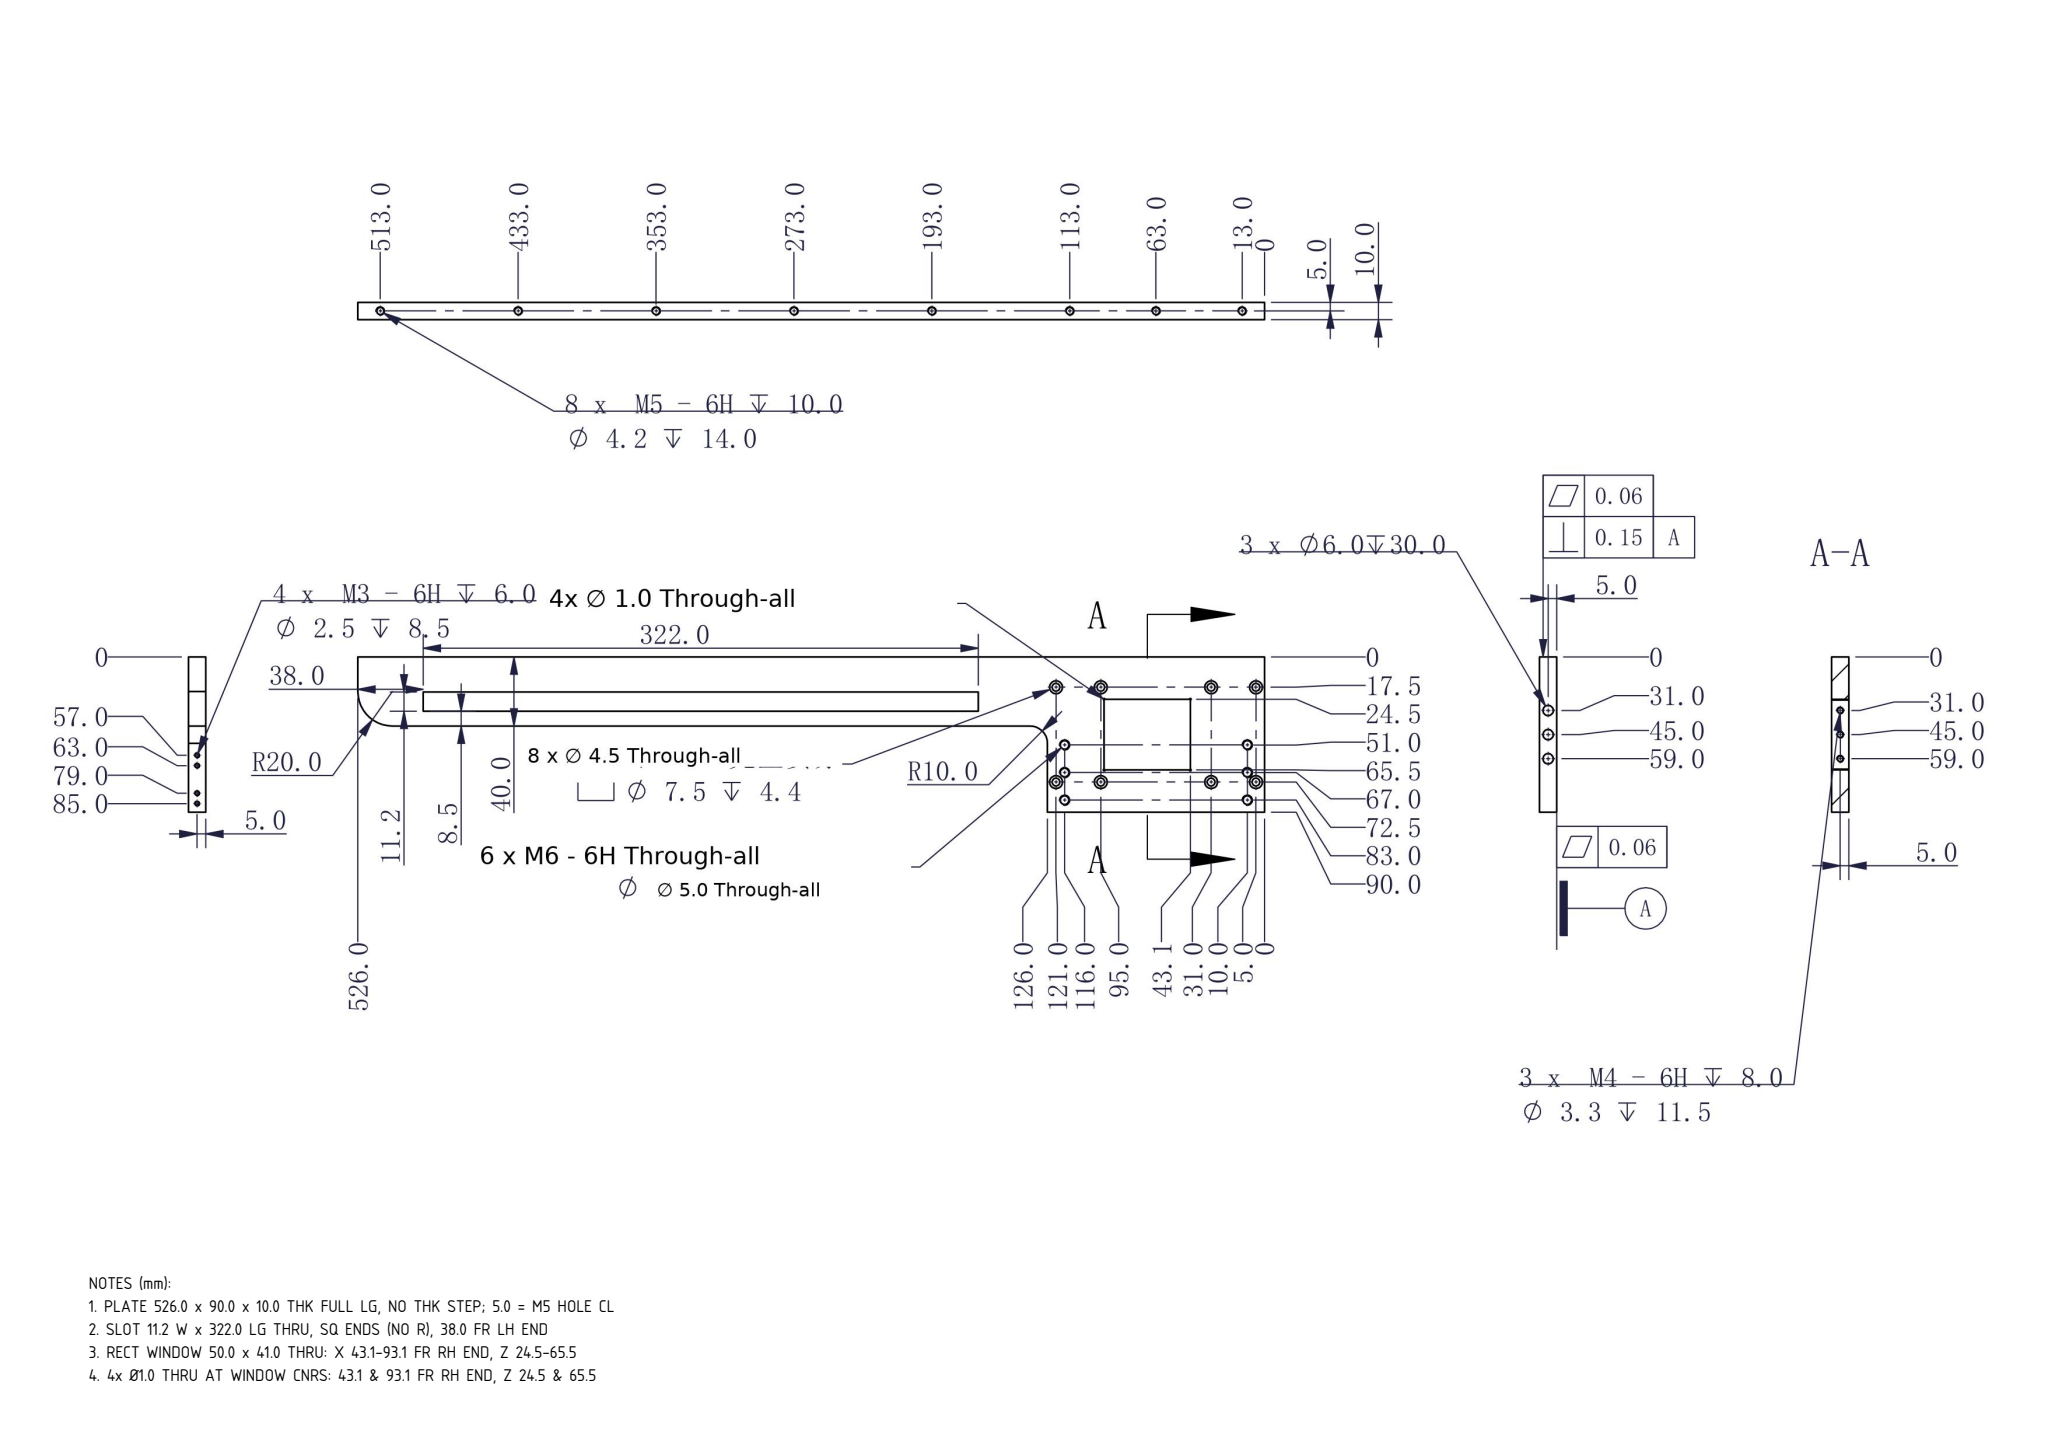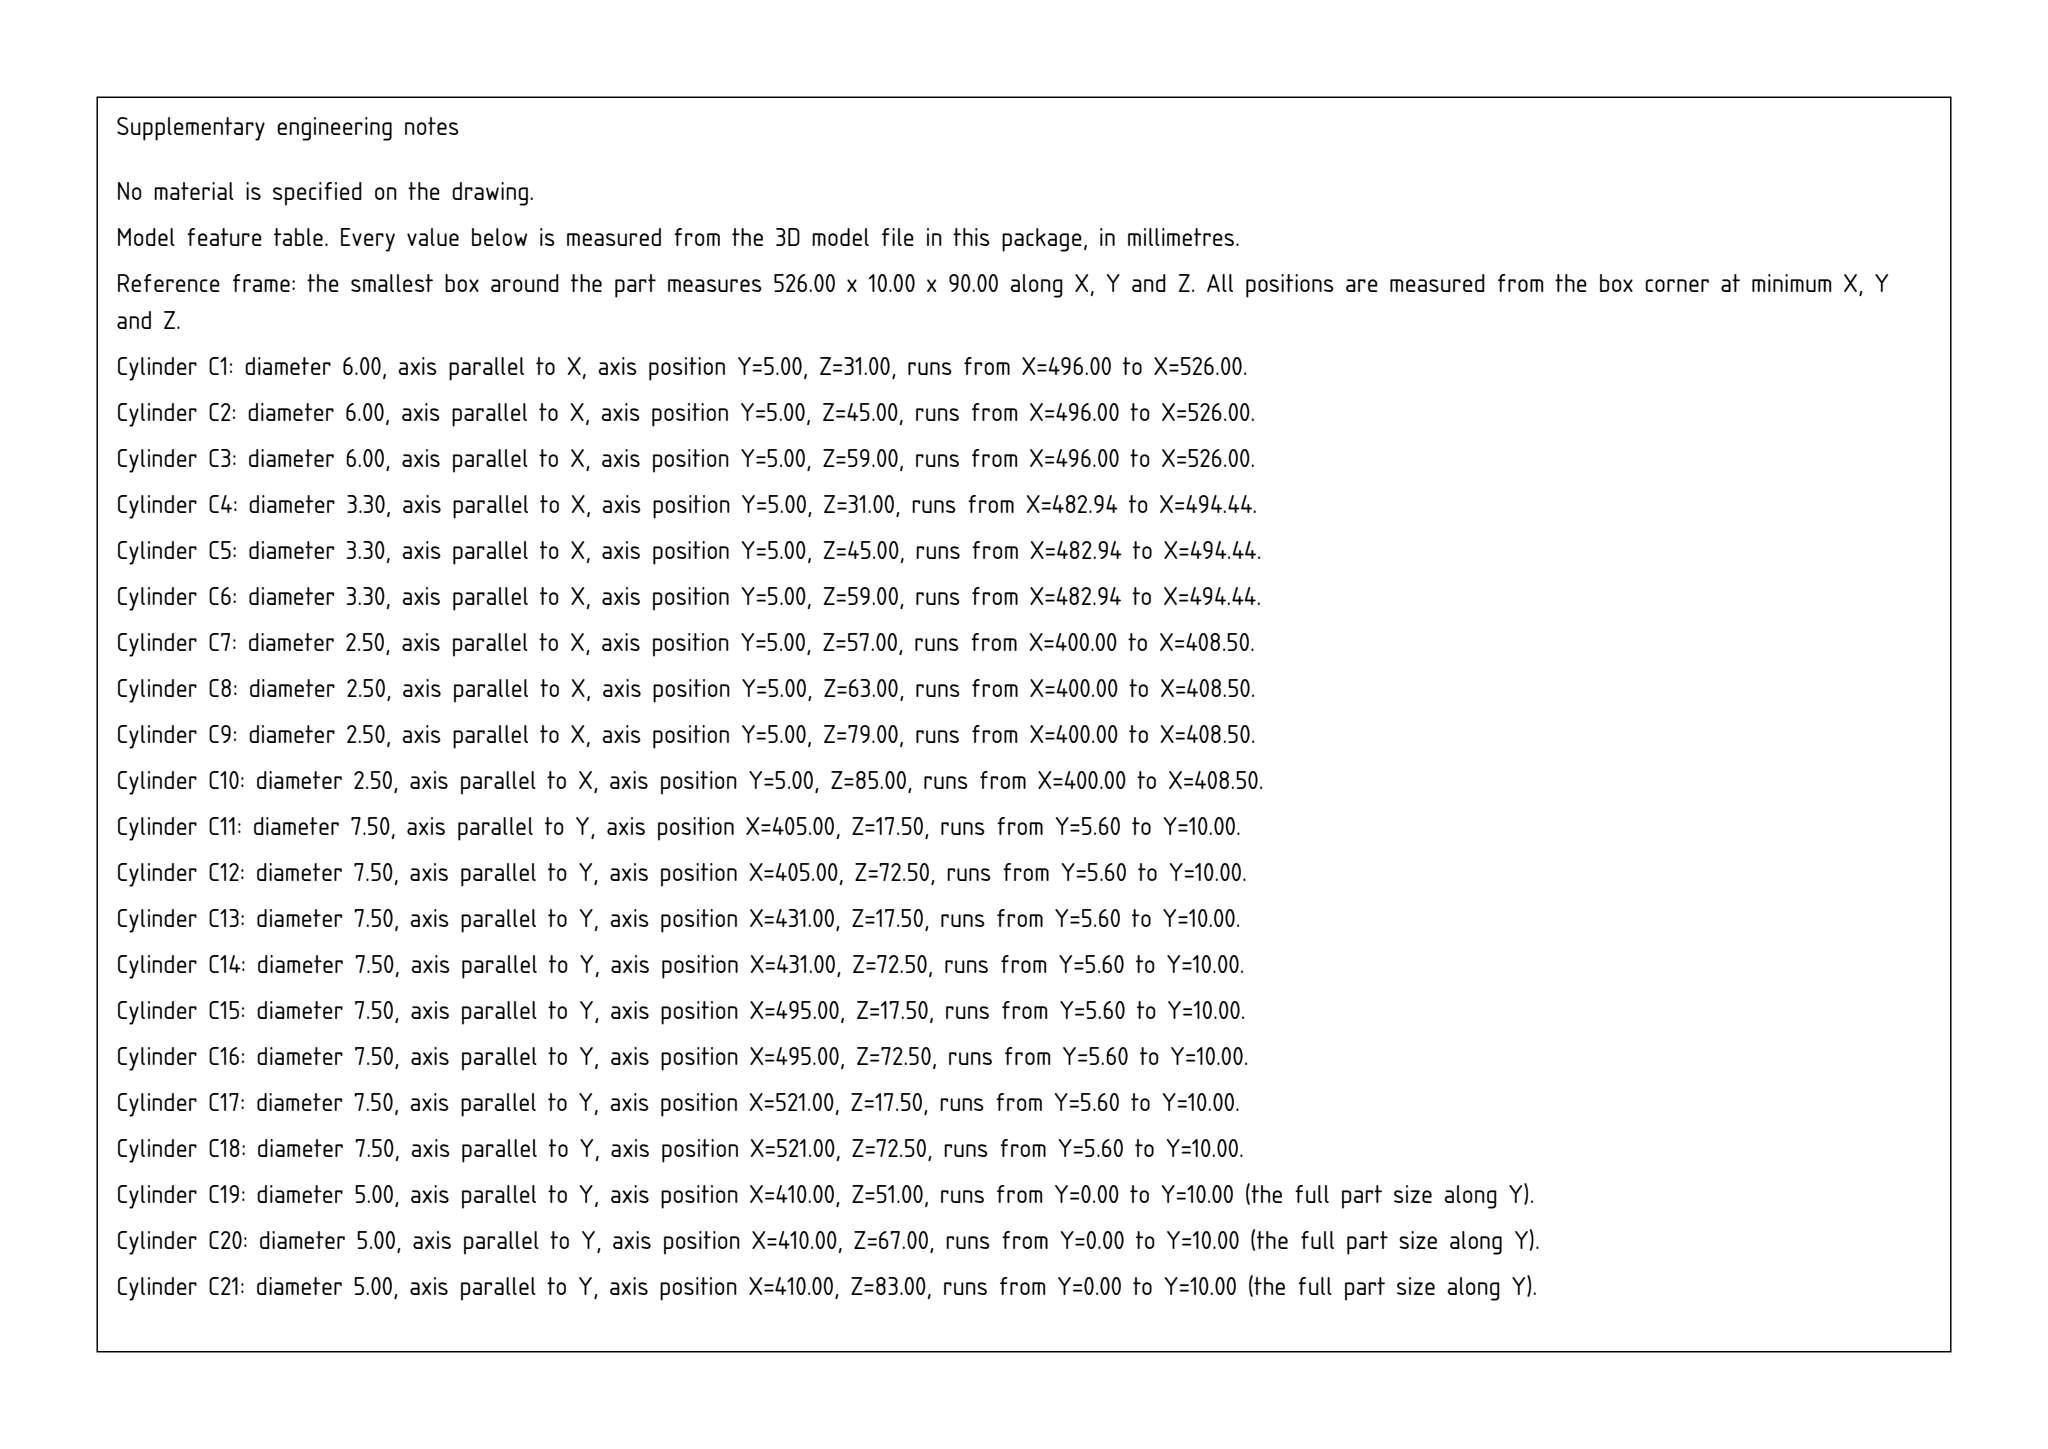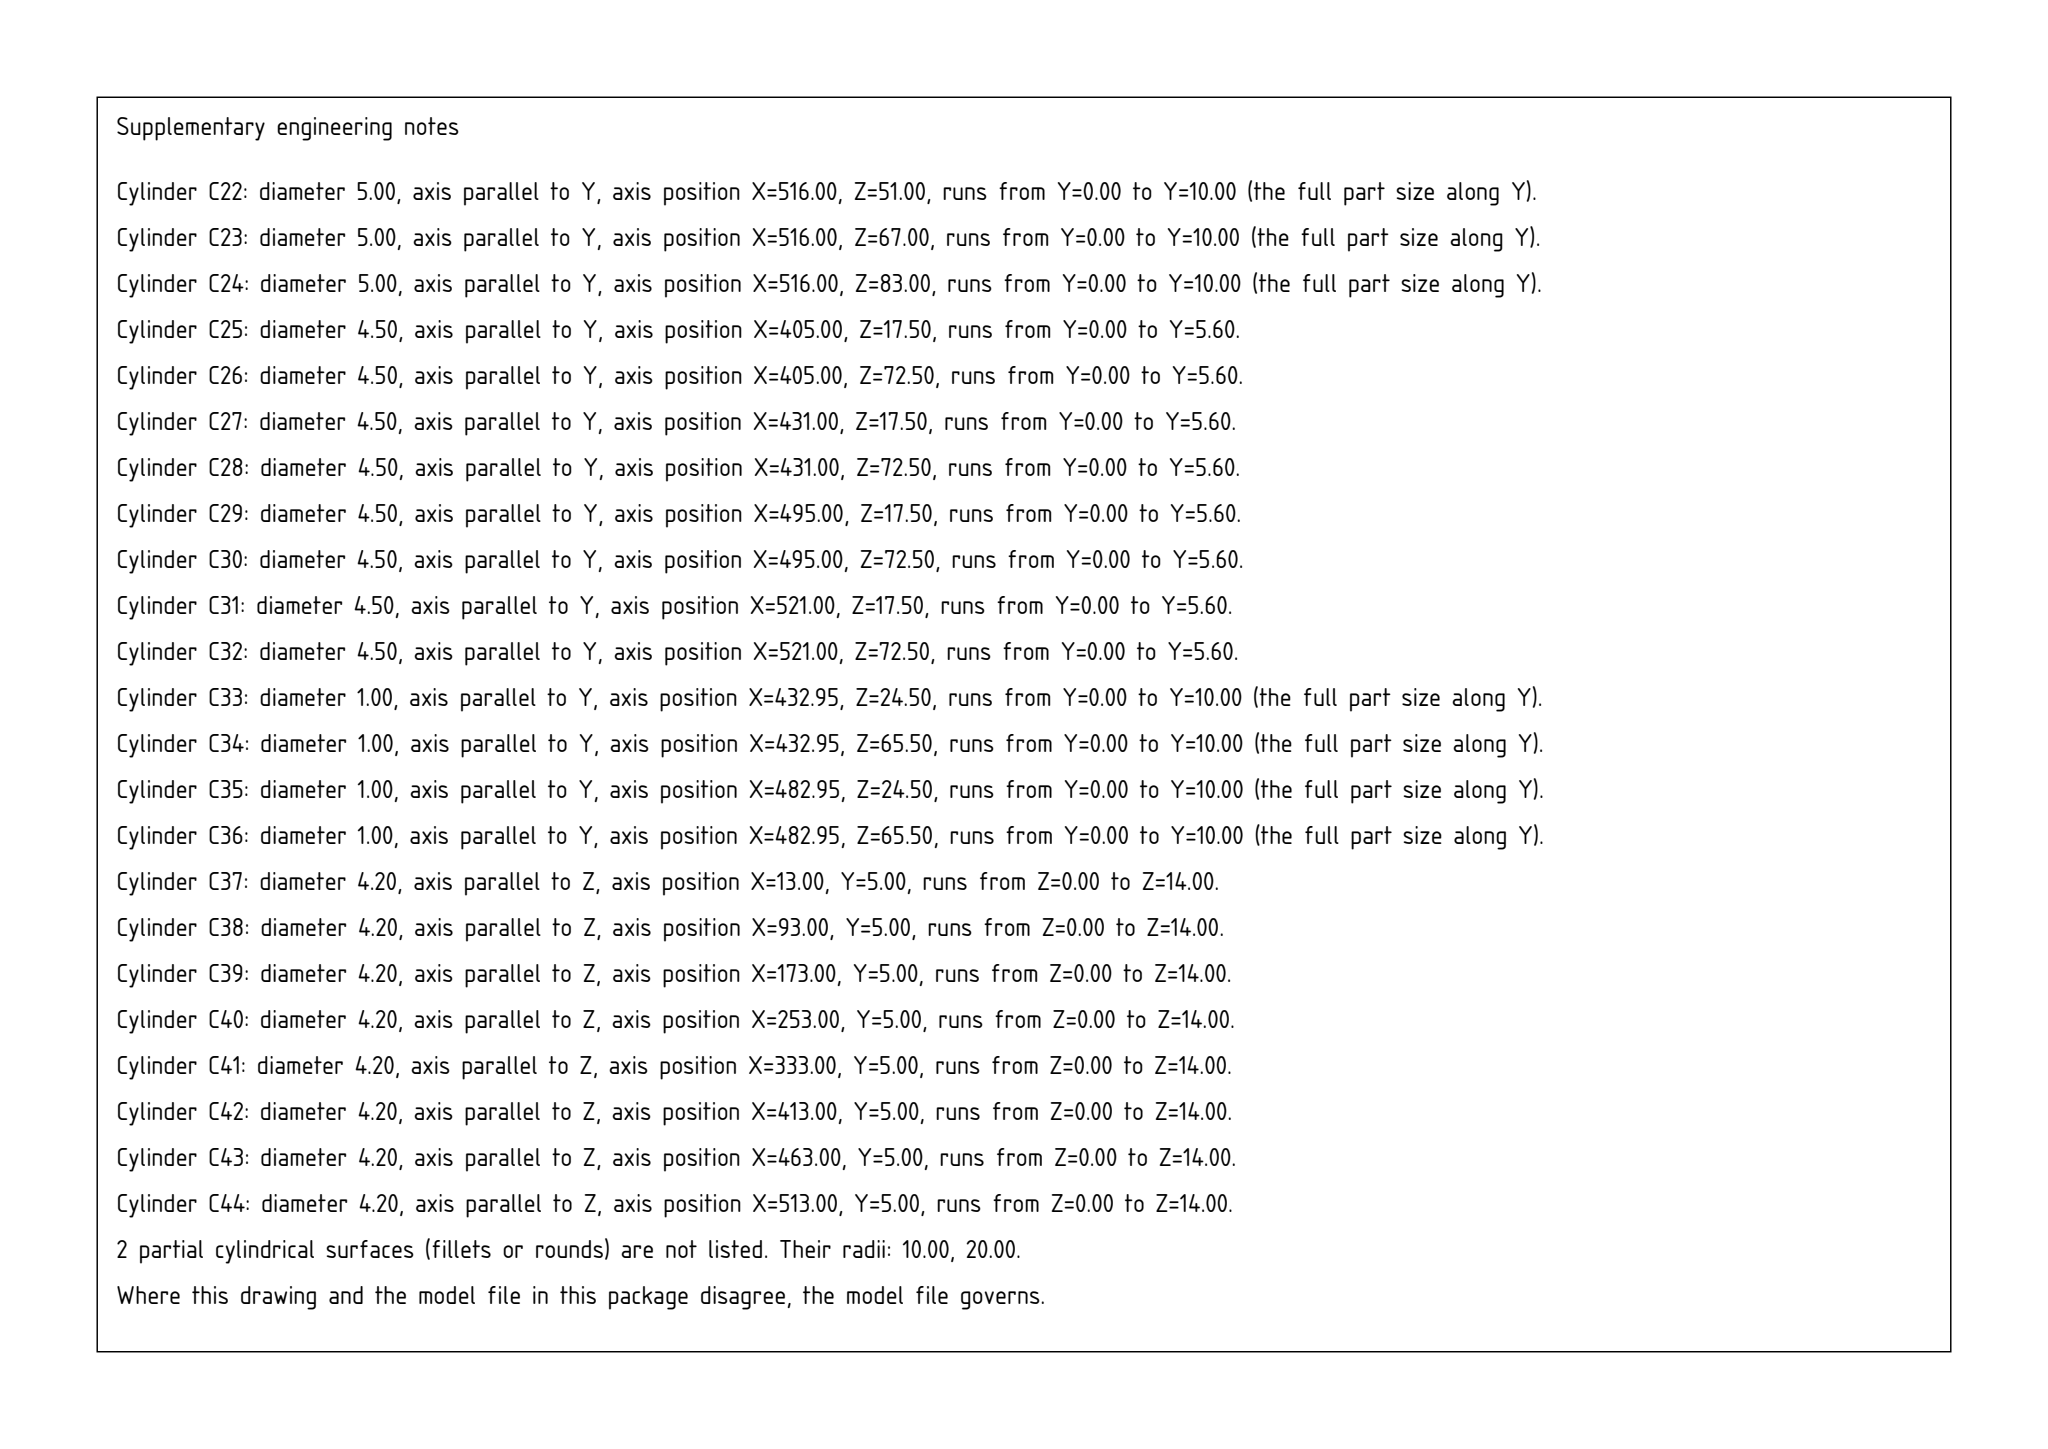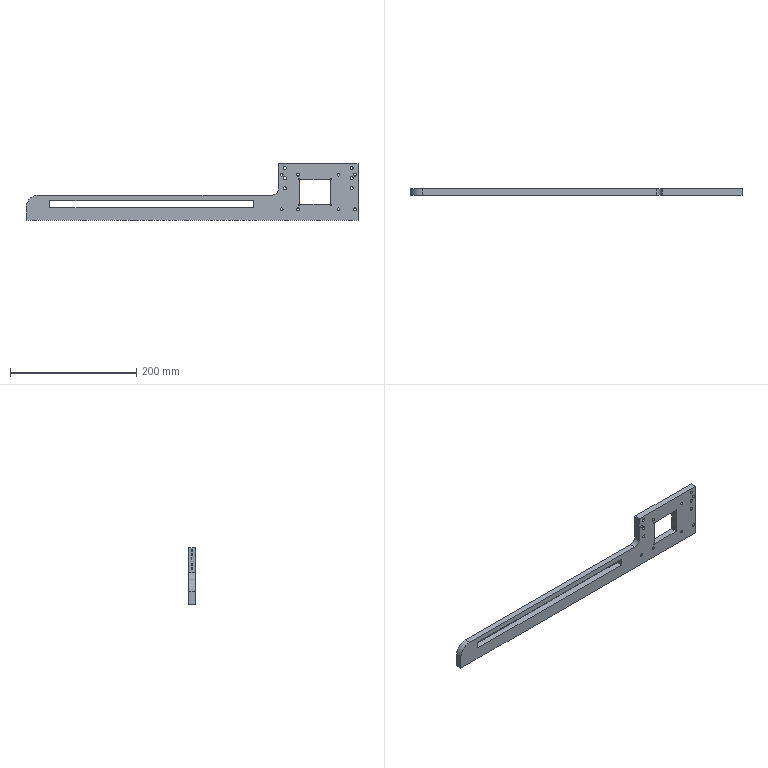Part | SolidWorks | mm | 1 solid | 145 faces | box 526 x 10 x 90 mm | volume 208164 mm3 | cylinder 88 | cone 30 | plane 27 | commonest cylinder face diameters 4.2 x16 7.5 x16 4.5 x16 5 x12 2.5 x8 6 x6 3.3 x6 1 x6
Drawing notes:
PLATE 526.0 x 90.0 x 10.0 THK FULL LG, NO THK STEP; 5.0 = M5 HOLE CL | from the solid: bbox 526x10x90; only y-planes 0.0 and 10.0 (y=5.6 are Ø7.5 CBORE floors); Ø4.2 M5 holes on y=5.0 CL
SLOT 11.2 W x 322.0 LG THRU, SQ ENDS (NO R), 38.0 FR LH END | from the solid: x-planes 37.98 & 359.97 (322.0 lg); z-planes 20.32 & 31.5 (11.18 w); y 0-10 thru; fillet_radii empty
RECT WINDOW 50.0 x 41.0 THRU: X 43.1-93.1 FR RH END, Z 24.5-65.5 | from the solid: x-planes 432.95/482.95 and z-planes 24.5/65.5 bound opening in end plate (x 400-526), 10.0 thru
4x Ø1.0 THRU AT WINDOW CNRS: 43.1 & 93.1 FR RH END, Z 24.5 & 65.5 | from the solid: Ø1.0 y-axis cyls at x=432.95 & 482.95, z=24.5 & 65.5, len 10.0; 50.0 apart
build123d program:
from build123d import *

# Parameters (mm, degrees)
SKETCH1_W                                       = 126
SKETCH1_H                                       = 10
BOSS_EXTRUDE1_DEPTH                             = 45
SKETCH2_W                                       = 50
SKETCH2_H                                       = 41
CUT_EXTRUDE1_DEPTH                              = 79.064
F_1_0_1_DIAMETER_HOLE1_D                        = 1
M4_TAPPED_HOLE1_D                               = 3.3
M4_TAPPED_HOLE1_DEPTH                           = 11.5
M4_TAPPED_HOLE1_TIP                             = 0.9914
M4_HEX_SOCKET_HEAD_CAP_SCREW_CBORE1_D           = 4.5
M4_HEX_SOCKET_HEAD_CAP_SCREW_CBORE1_CBORE_D     = 7.5
M4_HEX_SOCKET_HEAD_CAP_SCREW_CBORE1_CBORE_DEPTH = 4.4
LPATTERN1_COUNT                                 = 3
LPATTERN1_PITCH                                 = 50
M6_TAPPED_HOLE1_D                               = 5
M3_TAPPED_HOLE1_D                               = 2.5
M3_TAPPED_HOLE1_DEPTH                           = 8.5
M3_TAPPED_HOLE1_TIP                             = 0.7511
SKETCH16_W                                      = 40
SKETCH16_H                                      = 10
BOSS_EXTRUDE2_DEPTH                             = 400
FILLET1_R                                       = 20
FILLET2_R                                       = 10
LPATTERN2_COUNT                                 = 6
LPATTERN2_PITCH                                 = 80
SKETCH17_R                                      = 3
CUT_EXTRUDE2_DEPTH                              = 30
SKETCH18_W                                      = 321.995
SKETCH18_H                                      = 11.182
CUT_EXTRUDE3_DEPTH                              = 61


with BuildPart() as part:
    # Sketch1 → Boss-Extrude1 (new, symmetric)
    with BuildSketch(Plane.XY):
        Rectangle(SKETCH1_W, SKETCH1_H)
    extrude(amount=BOSS_EXTRUDE1_DEPTH, both=True)

    # Sketch2 → Cut-Extrude1 (cut, through all)
    with BuildSketch(Plane(origin=(0, 5, 0), x_dir=(1, 0, 0), z_dir=(0, 1, 0))):
        with Locations((-5.055, 0)):
            Rectangle(SKETCH2_W, SKETCH2_H)
    extrude(amount=-CUT_EXTRUDE1_DEPTH, mode=Mode.SUBTRACT)

    # 1.0 _1_ Diameter Hole1 (through all)
    with Locations(Plane.XZ.offset(5)):
        with Locations((-30.055, 20.5), (19.945, 20.5), (19.945, -20.5), (-30.055, -20.5)):
            Hole(F_1_0_1_DIAMETER_HOLE1_D / 2)

    # M4 Tapped Hole1
    with Locations(Plane.ZY.offset(-19.945)):
        with Locations((14, 0), (0, 0), (-14, 0)):
            Hole(M4_TAPPED_HOLE1_D / 2, depth=M4_TAPPED_HOLE1_DEPTH)
            with Locations((0, 0, -(M4_TAPPED_HOLE1_DEPTH + M4_TAPPED_HOLE1_TIP / 2))):  # 118° drill point
                Cone(0, M4_TAPPED_HOLE1_D / 2, M4_TAPPED_HOLE1_TIP, mode=Mode.SUBTRACT)

    # M4 Hex Socket Head Cap Screw CBORE1 (through all)
    with Locations(Plane(origin=(0, 5, 0), x_dir=(-1, 0, 0), z_dir=(0, 1, 0))):
        with Locations((-32, 27.5), (-58, 27.5), (-58, -27.5), (-32, -27.5), (32, -27.5), (58, -27.5), (58, 27.5), (32, 27.5)):
            CounterBoreHole(M4_HEX_SOCKET_HEAD_CAP_SCREW_CBORE1_D / 2, M4_HEX_SOCKET_HEAD_CAP_SCREW_CBORE1_CBORE_D / 2, M4_HEX_SOCKET_HEAD_CAP_SCREW_CBORE1_CBORE_DEPTH)

    # Sketch10 → M5 Tapped Hole1 (revolve, cut)
    with BuildSketch(Plane(origin=(-50, 0, -45), x_dir=(0, 1, 0), z_dir=(1, 0, 0))):
        Polygon((0, 0), (0, 15.262), (2.1, 14), (2.1, 0), align=None)
    m5_tapped_hole1 = revolve(axis=Axis((-50, 0, -51.35), (0, 0, 1)), mode=Mode.SUBTRACT)

    # LPattern1: M5 Tapped Hole1 ×3
    with Locations(*[(i * LPATTERN1_PITCH, 0, 0) for i in range(1, LPATTERN1_COUNT)]):
        add(m5_tapped_hole1, mode=Mode.SUBTRACT)

    # M6 Tapped Hole1 (through all)
    with Locations(Plane(origin=(0, 5, 0), x_dir=(1, 0, 0), z_dir=(0, 1, 0))):
        with Locations((53, -38), (53, -22), (53, -6), (-53, -38), (-53, -22), (-53, -6)):
            Hole(M6_TAPPED_HOLE1_D / 2)

    # M3 Tapped Hole1
    with Locations(Plane.ZY.offset(63)):
        with Locations((18, 0), (12, 0), (34, 0), (40, 0)):
            Hole(M3_TAPPED_HOLE1_D / 2, depth=M3_TAPPED_HOLE1_DEPTH)
            with Locations((0, 0, -(M3_TAPPED_HOLE1_DEPTH + M3_TAPPED_HOLE1_TIP / 2))):  # 118° drill point
                Cone(0, M3_TAPPED_HOLE1_D / 2, M3_TAPPED_HOLE1_TIP, mode=Mode.SUBTRACT)

    # Sketch16 → Boss-Extrude2 (add)
    with BuildSketch(Plane.ZY.offset(63)):
        with Locations((-25, 0)):
            Rectangle(SKETCH16_W, SKETCH16_H)
    extrude(amount=BOSS_EXTRUDE2_DEPTH)

    # Fillet1
    fillet1_edges = [part.edges().sort_by_distance(p)[0] for p in [
        (-463, 0, -5),
    ]]
    fillet(fillet1_edges, radius=FILLET1_R)

    # Fillet2
    fillet2_edges = [part.edges().sort_by_distance(p)[0] for p in [
        (-63, 0, -5),
    ]]
    fillet(fillet2_edges, radius=FILLET2_R)

    # LPattern2: M5 Tapped Hole1 ×6
    with Locations(*[(-i * LPATTERN2_PITCH, 0, 0) for i in range(1, LPATTERN2_COUNT)]):
        add(m5_tapped_hole1, mode=Mode.SUBTRACT)

    # Sketch17 → Cut-Extrude2 (cut)
    with BuildSketch(Plane(origin=(63, 0, 0), x_dir=(0, 0, -1), z_dir=(1, 0, 0))):
        with Locations((-14, 0)):
            Circle(SKETCH17_R)
        Circle(SKETCH17_R)
        with Locations((14, 0)):
            Circle(SKETCH17_R)
    extrude(amount=-CUT_EXTRUDE2_DEPTH, mode=Mode.SUBTRACT)

    # Sketch18 → Cut-Extrude3 (cut)
    with BuildSketch(Plane(origin=(0, 5, 0), x_dir=(1, 0, 0), z_dir=(0, 1, 0))):
        with Locations((-264.026, 19.092)):
            Rectangle(SKETCH18_W, SKETCH18_H)
    extrude(amount=-CUT_EXTRUDE3_DEPTH, mode=Mode.SUBTRACT)


solid = part.part